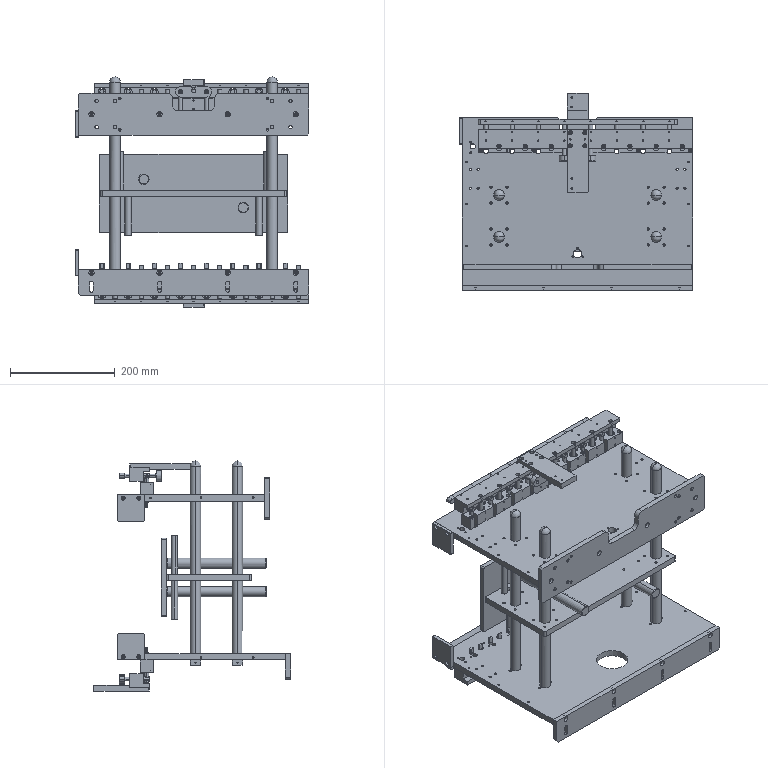Assembly | SolidWorks | mm | 81 component files | 81 solids | 2796 faces | box 446 x 377 x 439.5 mm | volume 6536936 mm3 | cylinder 1578 | plane 840 | cone 370 | sphere 8 | commonest cylinder face diameters 2.5 x358 8 x268 4.2 x160 3.3 x144 4.5 x124 10 x102 15 x64 5.5 x44
Bill of materials:
J-009 | 1 | 45 | Long rectangular bar split into a row of block segments by narrow U-shaped slots that open from one long side, with a large through hole and smaller holes in each segment.
J-010 | 16 | 45 | Cylindrical pin with a small axial hole in one end. The other end narrows to a flat, blade-like tang with an angled tip.
J-011 | 1 | 45 | Long bar with an L-shaped (rabbeted) cross-section. It has a row of larger holes, rows of small holes, and a U-notch in the middle of one long edge.
J-012 | 2 | 45 | Spool-shaped body with two coaxial flanges joined by a smaller-diameter hub, a central through bore, and a flat cut on the side of one flange.
J-013 | 1 | 45 | Long, slender flat bar with full-radius rounded ends and a single row of evenly spaced small through holes.
J-014 | 14 | 45 | Solid cylindrical pin with chamfered ends and a single radial cross-hole near one end, with local flats or recesses around it.
J-015 | 16 | 45 | Cylindrical pin with a small axial hole and flats at one end, and a narrower, flattened tang with an angled tip at the other end.
J-016 | 1 | 45 | Rectangular plate with small chamfered corners, a stepped underside, and a cluster of larger and small holes near one end plus two small holes near the other end.
J-017 | 2 | 45 | Tubular pin with an axial through bore, chamfered ends, and one radial cross-hole off-center with local relief cuts.
J-018 | 1 | 45 | Large thin rectangular plate with a rounded-corner rectangular notch in one edge and many holes: a row of alternating round holes and short slots, four large holes with surrounding small-hole patterns, a smaller hole pattern near the opposite edge, and edge holes.
J-002 | 1 | 45 | Flat link plate with full-radius ends, a through hole near each end, and a central round-ended slot open from one long edge with a stepped (wider at top) profile.
J-008 | 2 | 45 | Thick, nearly square flat plate with chamfered corners and two through holes near one edge.
J-020 | 1 | 45 | Long, thin rectangular flat plate. One long edge has a single wide rectangular notch with rounded corners at mid-length, and the plate has a pattern of through-holes that is roughly mirror-symmetric.
J-024 | 1 | 45 | Rectangular block-like plate whose top surface steps up in three levels along its length. The lowest end has a pattern of through-holes, and the highest end has two holes.
J-025 | 1 | 45 | Long, slender flat bar with fully rounded ends and a row of evenly spaced small holes. A raised central boss has a slot opening on one side and a stepped profile.
J-026 | 1 | 45 | Long, deep rectangular bar divided by repeated slots into eight block segments. Each segment has a large vertical through-bore, small holes on top, and two small holes on the side face. One central segment is raised above the others.
J-027 | 1 | 45 | Long bar with an L-shaped cross-section: a tall rib on a wider base flange. Eight large horizontal bores pass through the rib along its length, and there are rows of small holes on top. A notch interrupts the rib near mid-length.
J-001 | 1 | 45 | Large, thin rectangular plate with a rectangular notch with rounded corners in one long edge. It has a row of alternating round holes and elongated slots near that edge, four medium holes each with two small flanking holes, one large central circular opening, and scattered small holes.
J-003 | 4 | 45 | Slender cylindrical rod or pin with at least one rounded or domed end.
J-004 | 4 | 45 | Solid rectangular block with chamfered vertical corners and three vertical through-holes in a row. The middle hole is larger than the two outer holes.
J-019 | 1 | 45 | Long, flat rectangular bar with chamfered corners. Four evenly spaced stations each have a small round hole and a vertical elongated slot below it.
J-005 | 1 | 45 | Rectangular flat plate with slightly rounded corners. It has four large holes near the corners, each surrounded by four small holes, plus many small holes in roughly symmetric groups across the plate.
J-006 | 1 | 45 | Thin rectangular plate with slightly rounded corners and six small through-holes. Four sit on the central row, and two slightly larger holes are offset above and below the row.
J-007 | 2 | 45 | Plain solid cylindrical rod or pin with flat ends and small edge chamfers.
J-028 | 4 | 45 | Long, slender solid cylinder with a small chamfer or edge break at its ends and a central axial hole in at least one end face. The hole looks like a blind bore with a conical (drill-point-like) bottom. Rod or sleeve-like shape.
Mates:
1. coincident | J-005-1 face at (397.325, 258.019, 276.731) dir (0, 1, 0) | J-006-1 face at (220.325, 258.019, 270.731) dir (0, -1, 0)
2. coincident | J-007-1 face at (125.325, 258.019, 297.731) dir (0, 1, 0) | J-007-2 face at (315.325, 258.019, 243.731) dir (0, 1, 0)
3. concentric | J-005-1 face at (70.325, 258.019, 270.731) dir (0, 1, 0) r 2.1 | J-006-1 face at (70.325, 268.019, 270.731) dir (0, 1, 0) r 5
4. concentric | J-005-1 face at (270.325, 258.019, 270.731) dir (0, 1, 0) r 2.1 | J-006-1 face at (270.325, 268.019, 270.731) dir (0, 1, 0) r 5
5. coincident | J-005-1 face at (397.325, 258.019, 276.731) dir (0, 1, 0) | J-007-1 face at (125.325, 258.019, 297.731) dir (0, 1, 0)
6. coincident | J-028-1 face at (95.325, 243.019, 264.731) dir (0, 0, 1) | J-028-2 face at (345.325, 243.019, 264.731) dir (0, 0, 1)
7. coincident | J-005-1 face at (220.325, 177.019, 264.731) dir (0, 0, -1) | J-028-1 face at (95.325, 243.019, 264.731) dir (0, 0, 1)
8. concentric | J-005-1 face at (95.325, 243.019, 276.731) dir (0, 0, 1) r 2.75 | J-028-1 face at (95.325, 243.019, 190.731) dir (0, 0, 1) r 6
9. concentric | J-005-1 face at (345.325, 243.019, 276.731) dir (0, 0, 1) r 2.75 | J-028-2 face at (345.325, 243.019, 190.731) dir (0, 0, 1) r 6
10. coincident | J-028-3 face at (80.325, 243.019, 276.731) dir (0, 0, -1) | J-028-4 face at (360.325, 243.019, 276.731) dir (0, 0, -1)
11. coincident | J-005-1 face at (220.325, 177.019, 276.731) dir (0, 0, 1) | J-028-3 face at (80.325, 243.019, 276.731) dir (0, 0, -1)
12. concentric | J-005-1 face at (360.325, 243.019, 264.731) dir (0, 0, -1) r 3.3 | J-028-4 face at (360.325, 243.019, 350.731) dir (0, 0, -1) r 6
13. concentric | J-005-1 face at (80.325, 243.019, 264.731) dir (0, 0, -1) r 3.3 | J-028-3 face at (80.325, 243.019, 350.731) dir (0, 0, -1) r 6
14. concentric | 002MaterialPickingModuleB-1/J-003-4 face at (370.325, 123.019, 493.231) dir (0, 0, -1) r 10 | assembly face at (370.325, 123.019, 371.231) dir (0, 0, 1) r 10
15. concentric | 002MaterialPickingModuleB-1/J-003-1 face at (70.325, 203.019, 493.231) dir (0, 0, -1) r 10 | assembly face at (70.325, 203.019, 371.231) dir (0, 0, 1) r 16
16. distance | 002MaterialPickingModuleA-1/J-002-1 face at (220.325, 211.019, 416.231) dir (0, 0, -1) | 002MaterialPickingModuleB-1/J-001-1 face at (220.325, 191.019, 125.231) dir (0, 0, 1)
17. coincident | J-002-1 face at (203.828, 242.655, 319.989) dir (0, 0, 1) | J-008-1 face at (-16.172, 382.655, 319.989) dir (0, 0, 1)
18. coincident | J-002-1 face at (-16.172, 102.655, 319.989) dir (-1, 0, 0) | J-008-1 face at (-16.172, 357.655, 294.989) dir (1, 0, 0)
19. coincident | J-002-1 face at (423.828, 382.655, 319.989) dir (0, 1, 0) | J-008-1 face at (-16.172, 382.655, 319.989) dir (0, 1, 0)
20. coincident | J-002-1 face at (203.828, 242.655, 319.989) dir (0, 0, 1) | 004SidePlugModule-1/J-009-1 face at (423.828, 340.155, 319.989) dir (0, 0, -1)
21. parallel | J-002-1 face at (423.828, 382.655, 319.989) dir (0, 1, 0) | 004SidePlugModule-1/J-009-1 face at (203.828, 340.155, 331.989) dir (0, 1, 0)
22. coincident | J-002-1 face at (423.828, 102.655, 319.989) dir (0, -1, 0) | J-020-1 face at (203.828, 102.655, 313.989) dir (0, 1, 0)
23. coincident | J-002-1 face at (423.828, 102.655, 319.989) dir (1, 0, 0) | J-020-1 face at (423.828, 102.655, 353.989) dir (1, 0, 0)
24. width | J-020-1 face at (423.828, 102.655, 353.989) dir (0, 0, 1) | J-020-1 face at (423.828, 102.655, 273.989) dir (0, 0, -1) | J-002-1 face at (203.828, 242.655, 307.989) dir (0, 0, -1) | J-002-1 face at (203.828, 242.655, 319.989) dir (0, 0, 1)
25. coincident | J-002-1 face at (423.828, 102.655, 319.989) dir (1, 0, 0) | 004SidePlugModule-1/J-009-1 face at (423.828, 340.155, 343.989) dir (1, 0, 0)
26. concentric | J-011-1 face at (181.119, 255.387, 367.448) dir (0, 0, -1) r 5 | J-012-1 face at (181.119, 255.387, 367.448) dir (0, 0, 1) r 5
27. concentric | J-015-1 face at (6.119, 232.387, 291.048) dir (0, 0, 1) r 4 | J-014-2 face at (6.119, 232.387, 359.448) dir (0, 0, 1) r 2.25
28. coincident | J-015-1 face at (6.119, 232.387, 349.448) dir (0, 0, 1) | J-014-2 face at (6.119, 274.387, 349.448) dir (0, 0, -1)
29. parallel | J-015-1 face at (2.655, 234.387, 301.048) dir (0, 1, 0) | J-014-2 face at (6.119, 226.387, 351.448) dir (0, -1, 0)
30. concentric | J-009-1 face at (6.119, 232.387, 314.948) dir (0, 0, 1) r 4.05 | J-015-1 face at (6.119, 232.387, 291.048) dir (0, 0, 1) r 4
31. coincident | J-011-1 face at (181.119, 255.387, 363.448) dir (0, 0, 1) | J-012-1 face at (173.44, 257.628, 363.448) dir (0, 0, -1)
32. coincident | J-014-2 face at (6.119, 274.387, 351.448) dir (0, 1, 0) | J-013-2 face at (181.119, 274.387, 351.448) dir (0, -1, 0)
33. concentric | J-014-2 face at (6.119, 226.387, 351.448) dir (0, 1, 0) r 4 | J-013-2 face at (6.119, 284.387, 351.448) dir (0, 1, 0) r 2.25
34. coincident | J-017-1 face at (156.119, 274.387, 349.448) dir (0, 0, -1) | J-015-9 face at (156.119, 232.387, 349.448) dir (0, 0, 1)
35. parallel | J-017-1 face at (148.619, 235.387, 349.448) dir (0, -1, 0) | J-015-9 face at (153.474, 229.387, 346.448) dir (0, -1, 0)
36. concentric | J-017-1 face at (156.119, 232.387, 359.448) dir (0, 0, 1) r 2.25 | J-015-9 face at (156.119, 232.387, 291.048) dir (0, 0, 1) r 4
37. coincident | J-013-2 face at (181.119, 274.387, 351.448) dir (0, -1, 0) | J-017-1 face at (156.119, 274.387, 351.448) dir (0, 1, 0)
38. parallel | J-010-4 face at (181.119, 232.387, 291.049) dir (0, 0, -1) | J-015-9 face at (156.119, 232.387, 291.048) dir (0, 0, -1)
39. coincident | J-017-1 face at (156.119, 214.387, 351.448) dir (0, -1, 0) | J-018-1 face at (156.119, 214.387, 351.448) dir (0, 1, 0)
40. concentric | J-017-1 face at (156.119, 214.387, 351.448) dir (0, -1, 0) r 1.65 | J-018-1 face at (156.119, 204.387, 351.448) dir (0, -1, 0) r 4
41. concentric | J-017-2 face at (206.119, 214.387, 351.448) dir (0, -1, 0) r 1.65 | J-018-1 face at (206.119, 204.387, 351.448) dir (0, -1, 0) r 4
42. coincident | J-011-1 face at (181.119, 245.887, 367.448) dir (0, 0, 1) | J-016-2 face at (181.119, 204.387, 367.448) dir (0, 0, -1)
43. coincident | J-011-1 face at (401.119, 227.387, 367.448) dir (0, -1, 0) | J-016-2 face at (201.119, 227.387, 367.448) dir (0, 1, 0)
44. coincident | 004SidePlugModule face at (381.119, 232.387, 359.448) dir (0, 0, 1) | J-011-1 face at (181.119, 245.887, 359.448) dir (0, 0, -1)
45. concentric | J-011-1 face at (167.119, 233.387, 367.448) dir (0, 0, 1) r 1.65 | J-016-2 face at (167.119, 233.387, 374.448) dir (0, 0, 1) r 2.25
46. concentric | J-009-1 face at (31.119, 232.387, 314.948) dir (0, 0, 1) r 7.5 | J-010-1 face at (31.119, 232.387, 291.049) dir (0, 0, 1) r 4
47. coincident | J-003-3 face at (392.106, 245.715, 293.864) dir (0, 0, -1) | J-003-4 face at (392.106, 165.715, 293.864) dir (0, 0, -1)
48. coincident | J-003-2 face at (92.106, 165.715, 293.864) dir (0, 0, -1) | J-003-3 face at (392.106, 245.715, 293.864) dir (0, 0, -1)
49. coincident | J-003-1 face at (92.106, 245.715, 293.864) dir (0, 0, -1) | J-003-2 face at (92.106, 165.715, 293.864) dir (0, 0, -1)
50. concentric | J-001-1 face at (92.106, 245.715, 293.864) dir (0, 0, -1) r 10 | J-003-1 face at (92.106, 245.715, 673.864) dir (0, 0, -1) r 10
51. concentric | J-001-1 face at (92.106, 165.715, 293.864) dir (0, 0, -1) r 10 | J-003-2 face at (92.106, 165.715, 673.864) dir (0, 0, -1) r 10
52. concentric | J-001-1 face at (392.106, 245.715, 293.864) dir (0, 0, -1) r 10 | J-003-3 face at (392.106, 245.715, 673.864) dir (0, 0, -1) r 10
53. concentric | J-001-1 face at (392.106, 165.715, 293.864) dir (0, 0, -1) r 10 | J-003-4 face at (392.106, 165.715, 673.864) dir (0, 0, -1) r 10
54. coincident | J-001-1 face at (242.106, 233.715, 293.864) dir (0, 0, -1) | J-003-3 face at (392.106, 245.715, 293.864) dir (0, 0, -1)
55. coincident | J-004-3 face at (392.106, 245.715, 293.864) dir (0, 0, 1) | J-004-4 face at (392.106, 165.715, 293.864) dir (0, 0, 1)
56. coincident | J-004-2 face at (92.106, 165.715, 293.864) dir (0, 0, 1) | J-004-3 face at (392.106, 245.715, 293.864) dir (0, 0, 1)
57. coincident | J-004-1 face at (92.106, 245.715, 293.864) dir (0, 0, 1) | J-004-2 face at (92.106, 165.715, 293.864) dir (0, 0, 1)
58. coincident | J-001-1 face at (242.106, 233.715, 293.864) dir (0, 0, -1) | J-004-1 face at (92.106, 245.715, 293.864) dir (0, 0, 1)
59. concentric | J-004-1 face at (92.106, 245.715, 283.864) dir (0, 0, -1) r 5.5 | J-003-1 face at (92.106, 245.715, 293.864) dir (0, 0, -1) r 3.4
60. concentric | J-003-2 face at (92.106, 165.715, 293.864) dir (0, 0, -1) r 3.4 | J-004-2 face at (92.106, 165.715, 283.864) dir (0, 0, -1) r 5.5
61. concentric | J-003-4 face at (392.106, 165.715, 293.864) dir (0, 0, -1) r 3.4 | J-004-4 face at (392.106, 165.715, 283.864) dir (0, 0, -1) r 3.3
62. concentric | J-003-3 face at (392.106, 245.715, 293.864) dir (0, 0, -1) r 3.4 | J-004-3 face at (392.106, 245.715, 283.864) dir (0, 0, -1) r 5.5
63. concentric | J-001-1 face at (406.106, 245.715, 293.864) dir (0, 0, -1) r 2.1 | J-004-3 face at (406.106, 245.715, 283.864) dir (0, 0, -1) r 2.75
64. concentric | J-001-1 face at (406.106, 165.715, 293.864) dir (0, 0, -1) r 2.1 | J-004-4 face at (406.106, 165.715, 283.864) dir (0, 0, -1) r 2.75
65. concentric | J-001-1 face at (106.106, 165.715, 293.864) dir (0, 0, -1) r 2.1 | J-004-2 face at (106.106, 165.715, 283.864) dir (0, 0, -1) r 2.75
66. concentric | J-001-1 face at (106.106, 245.715, 293.864) dir (0, 0, -1) r 2.1 | J-004-1 face at (106.106, 245.715, 283.864) dir (0, 0, -1) r 2.75
67. coincident | J-001-1 face at (22.106, 73.715, 305.864) dir (-1, 0, 0) | J-008-1 face at (22.106, 368.715, 318.864) dir (1, 0, 0)
68. coincident | J-001-1 face at (242.106, 233.715, 293.864) dir (0, 0, -1) | J-008-1 face at (22.106, 343.715, 293.864) dir (0, 0, -1)
69. coincident | J-001-1 face at (462.106, 393.715, 305.864) dir (0, 1, 0) | J-008-1 face at (22.106, 393.715, 293.864) dir (0, 1, 0)
70. coincident | J-001-1 face at (242.106, 233.715, 293.864) dir (0, 0, -1) | 004SidePlugModuleB-1/J-026-2 face at (22.106, 351.215, 293.864) dir (0, 0, 1)
71. distance | 004SidePlugModuleB-1/J-026-2 face at (242.106, 351.215, 281.864) dir (0, 1, 0) | J-001-1 face at (462.106, 393.715, 305.864) dir (0, 1, 0)
72. coincident | J-001-1 face at (462.106, 73.715, 305.864) dir (0, -1, 0) | J-019-1 face at (242.106, 73.715, 280.864) dir (0, 1, 0)
73. coincident | J-001-1 face at (242.106, 233.715, 305.864) dir (0, 0, 1) | J-019-1 face at (462.106, 73.715, 305.864) dir (0, 0, 1)
74. coincident | J-001-1 face at (22.106, 73.715, 305.864) dir (-1, 0, 0) | J-019-1 face at (22.106, 73.715, 305.864) dir (-1, 0, 0)
75. coincident | J-001-1 face at (462.106, 73.715, 305.864) dir (1, 0, 0) | 004SidePlugModuleB-1/J-026-2 face at (462.106, 351.215, 269.864) dir (1, 0, 0)
76. concentric | J-027-2 face at (181.119, 255.387, 367.448) dir (0, 0, -1) r 5 | J-012-1 face at (181.119, 255.387, 367.448) dir (0, 0, 1) r 5
77. concentric | J-015-1 face at (6.119, 232.387, 291.048) dir (0, 0, 1) r 4 | J-014-2 face at (6.119, 232.387, 359.448) dir (0, 0, 1) r 2.25
78. coincident | J-015-1 face at (6.119, 232.387, 349.448) dir (0, 0, 1) | J-014-2 face at (6.119, 274.387, 349.448) dir (0, 0, -1)
79. parallel | J-015-1 face at (2.655, 234.387, 301.048) dir (0, 1, 0) | J-014-2 face at (6.119, 226.387, 351.448) dir (0, -1, 0)
80. concentric | J-026-2 face at (6.119, 232.387, 314.948) dir (0, 0, 1) r 4.05 | J-015-1 face at (6.119, 232.387, 291.048) dir (0, 0, 1) r 4
81. coincident | J-027-2 face at (181.119, 255.387, 363.448) dir (0, 0, 1) | J-012-1 face at (173.44, 257.628, 363.448) dir (0, 0, -1)
82. coincident | J-014-2 face at (6.119, 274.387, 351.448) dir (0, 1, 0) | J-025-2 face at (181.119, 274.387, 351.448) dir (0, -1, 0)
83. concentric | J-014-2 face at (6.119, 226.387, 351.448) dir (0, 1, 0) r 4 | J-025-2 face at (6.119, 284.387, 351.448) dir (0, 1, 0) r 2.25
84. coincident | 004SidePlugModuleB face at (381.119, 232.387, 359.448) dir (0, 0, 1) | J-027-2 face at (181.119, 245.887, 359.448) dir (0, 0, -1)
85. coincident | J-027-2 face at (181.119, 245.887, 367.448) dir (0, 0, 1) | J-024-3 face at (181.119, 280.887, 367.448) dir (0, 0, -1)
86. concentric | J-027-2 face at (195.119, 233.387, 367.448) dir (0, 0, 1) r 1.65 | J-024-3 face at (195.119, 233.387, 374.448) dir (0, 0, 1) r 2.25
87. concentric | J-027-2 face at (167.119, 233.387, 367.448) dir (0, 0, 1) r 1.65 | J-024-3 face at (167.119, 233.387, 374.448) dir (0, 0, 1) r 2.25
88. coincident | J-010-1 face at (-18.881, 232.387, 359.448) dir (0, 0, 1) | J-027-2 face at (181.119, 245.887, 359.448) dir (0, 0, -1)